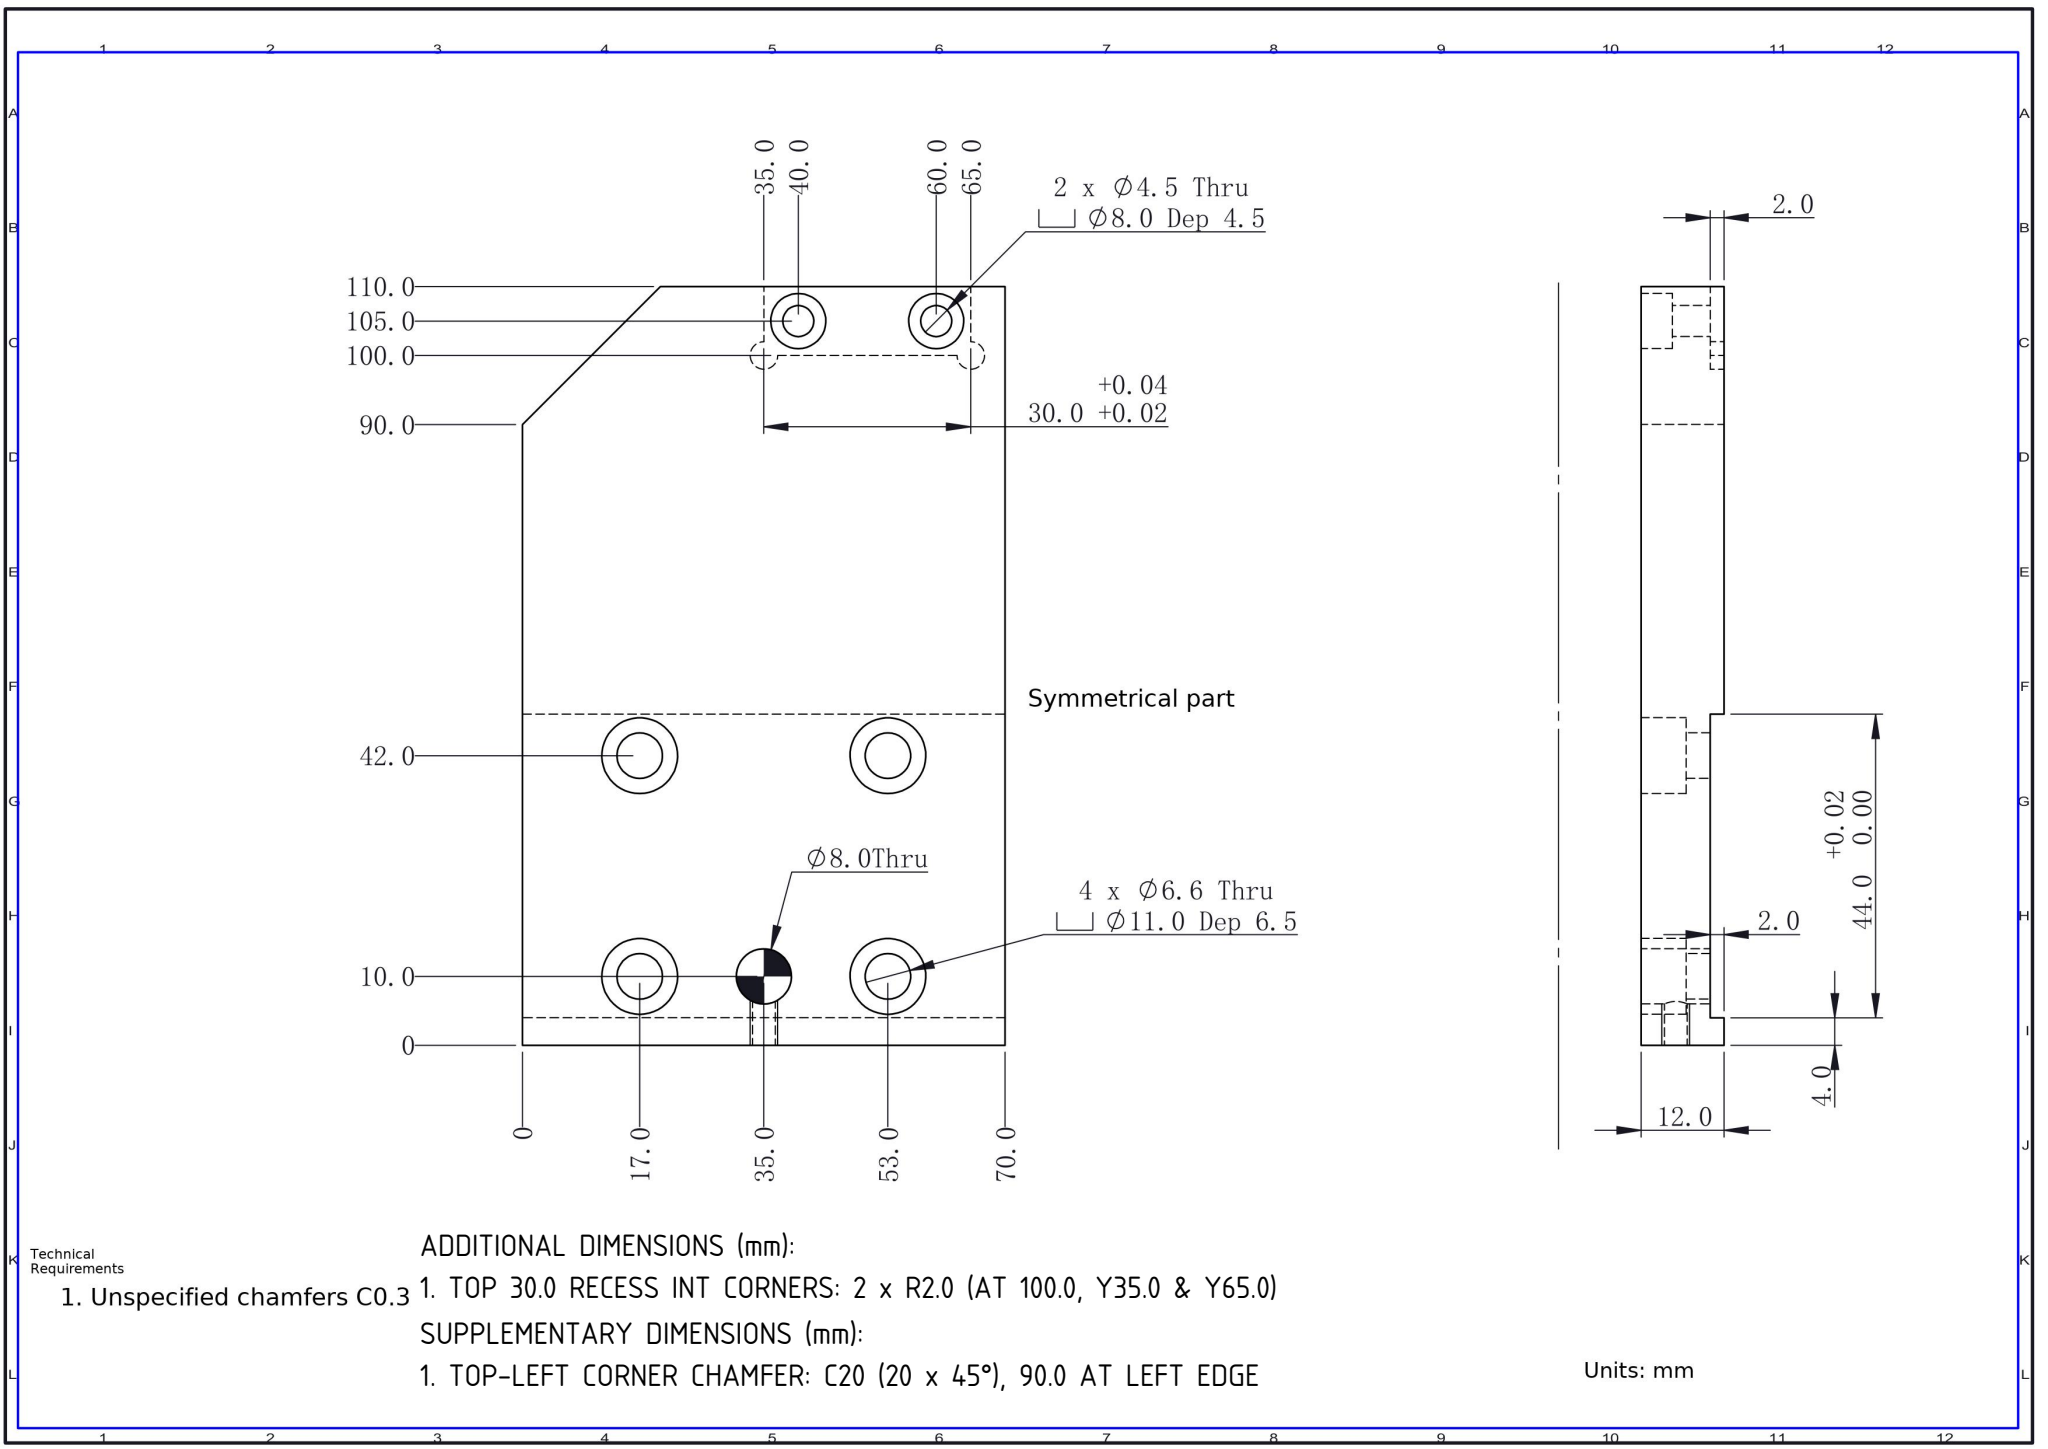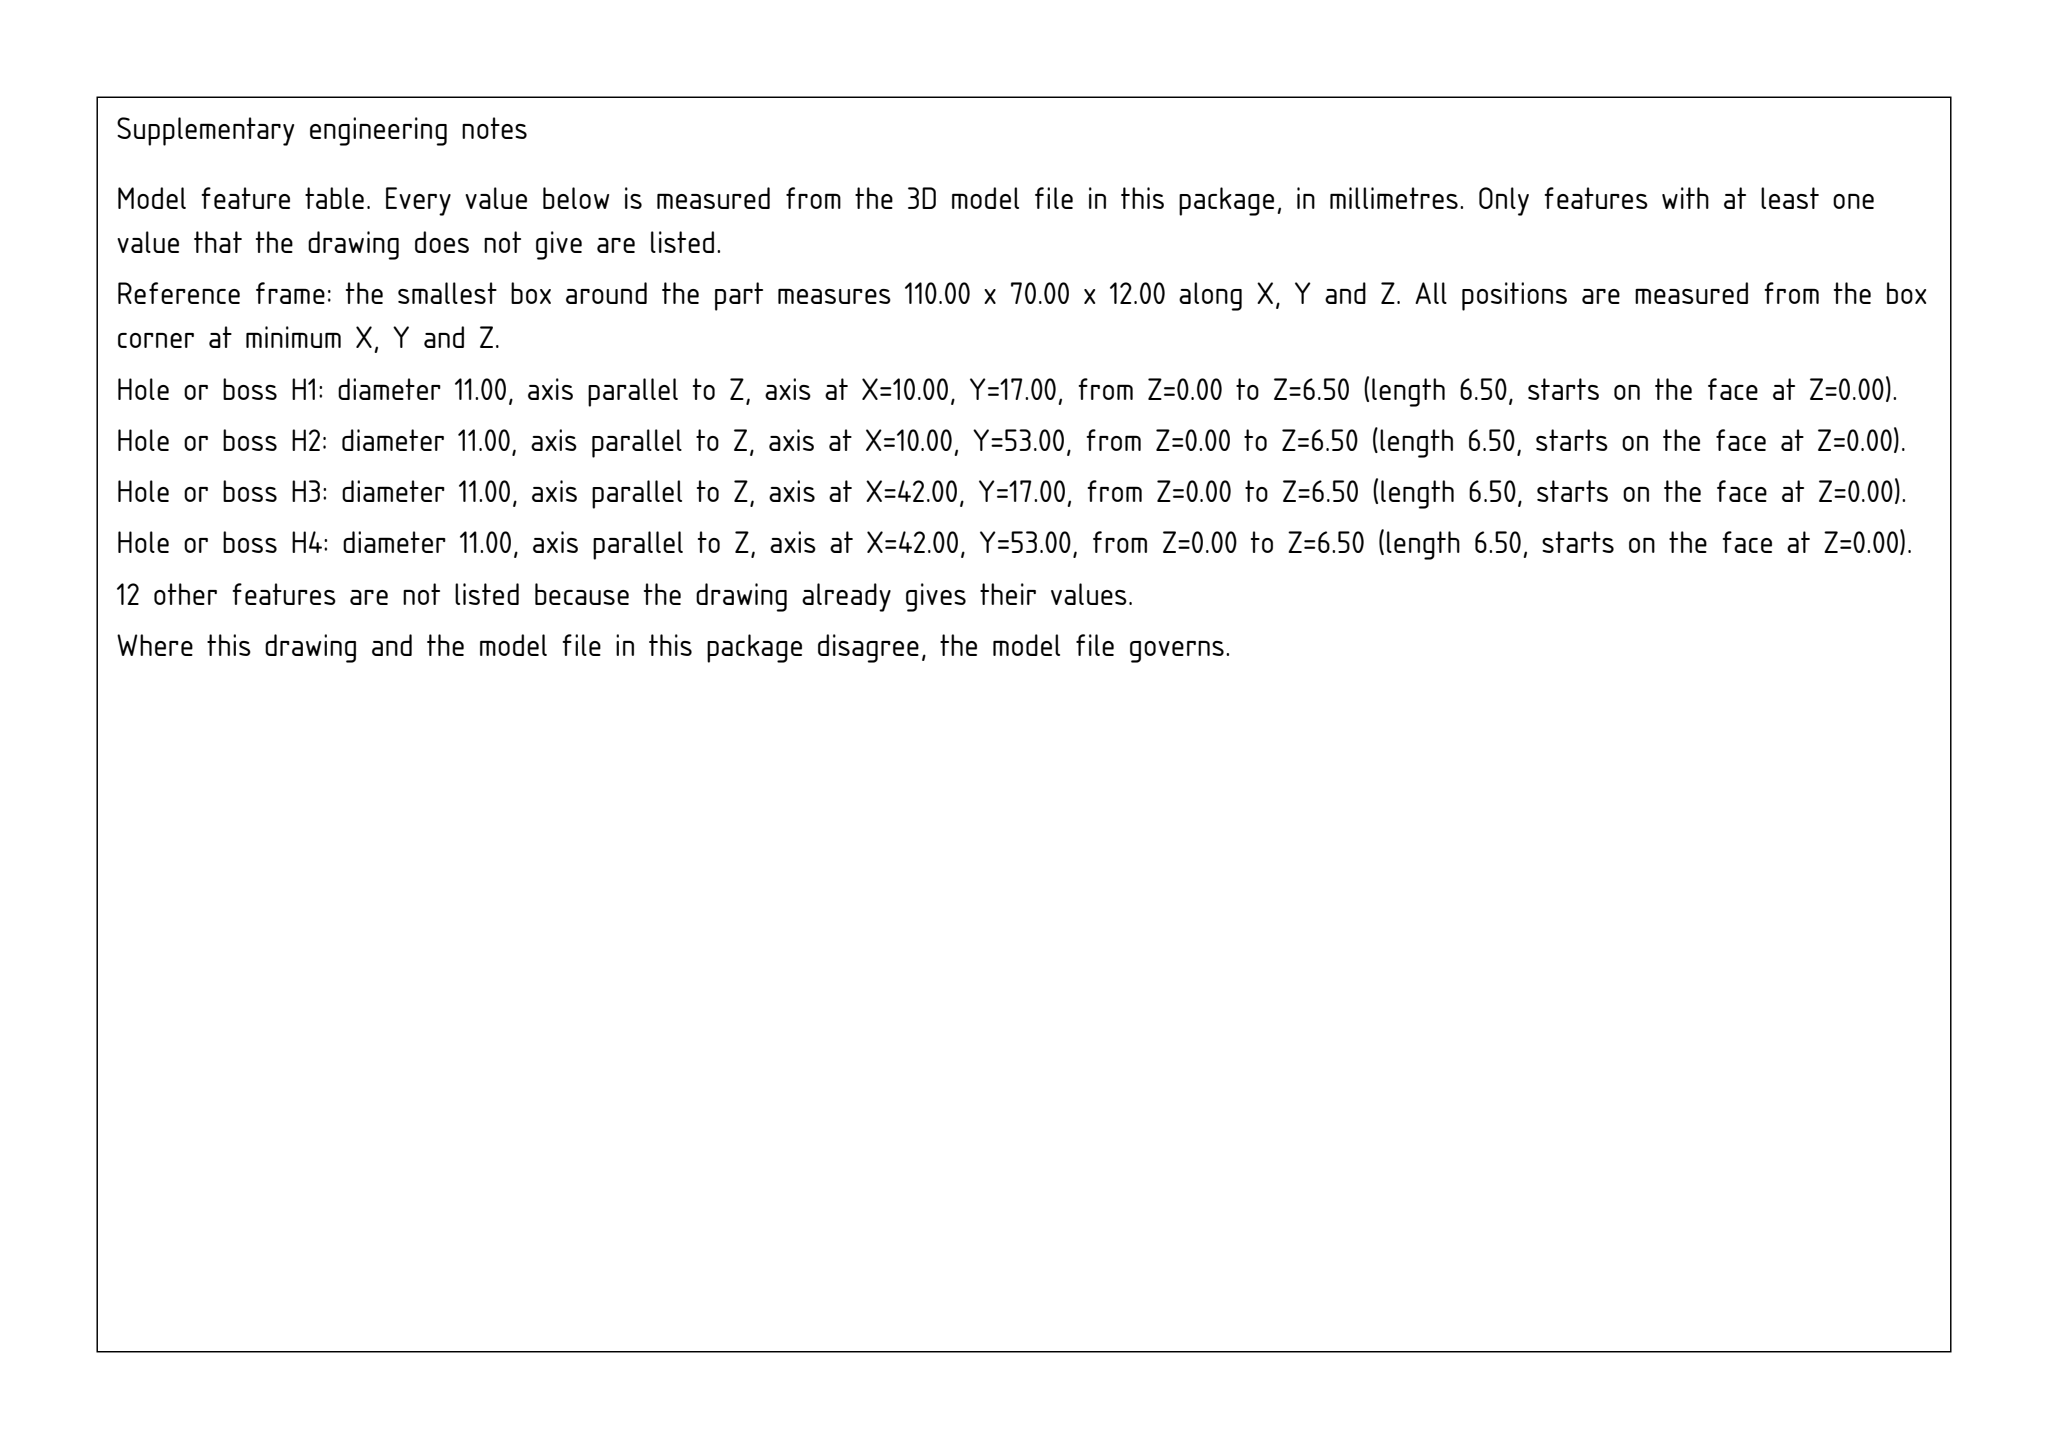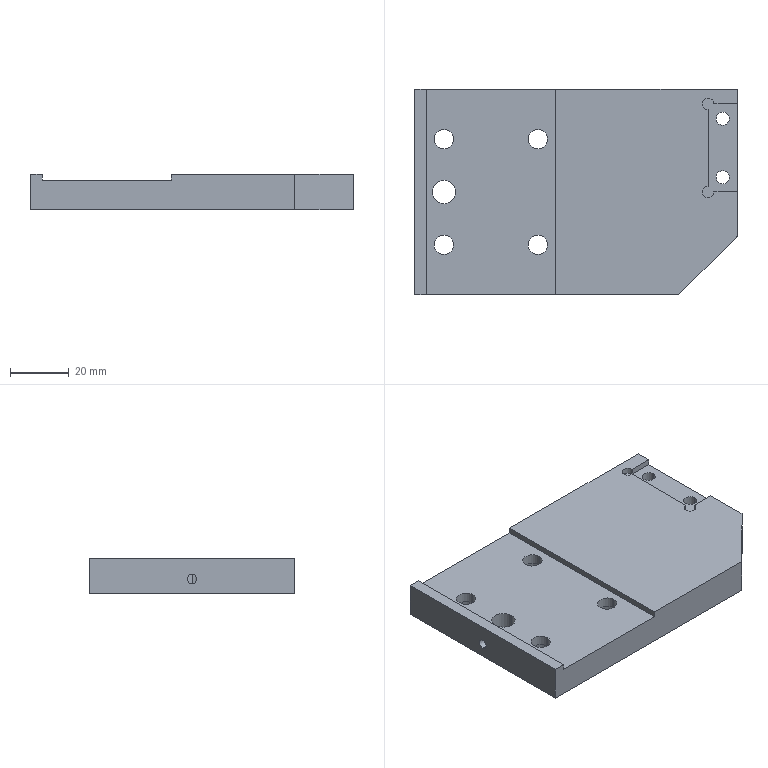Part | SolidWorks | mm | 1 solid | 51 faces | box 110 x 70 x 12 mm | volume 79070 mm3 | cylinder 30 | plane 21 | commonest cylinder face diameters 11 x8 6.6 x8 8 x6 4.5 x4 3.3 x2 4 x2
build123d program:
from build123d import *

# Parameters (mm, degrees)
SKETCH1_W                                       = 110
SKETCH1_H                                       = 70
BOSS_EXTRUDE1_DEPTH                             = 12
M6_HEX_SOCKET_HEAD_CAP_SCREW_CBORE1_D           = 6.6
M6_HEX_SOCKET_HEAD_CAP_SCREW_CBORE1_CBORE_D     = 11
M6_HEX_SOCKET_HEAD_CAP_SCREW_CBORE1_CBORE_DEPTH = 6.5
SKETCH6_W                                       = 44
SKETCH6_H                                       = 70
CUT_EXTRUDE1_DEPTH                              = 2
SIZE_MM_DOWEL_PIN_HOLE1_D                       = 8
SKETCH15_W                                      = 10
SKETCH15_H                                      = 30
CUT_EXTRUDE2_DEPTH                              = 2
SKETCH16_R                                      = 2
CUT_EXTRUDE3_DEPTH                              = 2
M4_HEX_SOCKET_HEAD_CAP_SCREW_CBORE1_D           = 4.5
M4_HEX_SOCKET_HEAD_CAP_SCREW_CBORE1_CBORE_D     = 8
M4_HEX_SOCKET_HEAD_CAP_SCREW_CBORE1_CBORE_DEPTH = 4.5
M4_TAPPED_HOLE1_REACH                           = 118.056
M4_TAPPED_HOLE1_BORE_R                          = 1.65
CHAMFER1_SIZE                                   = 20


with BuildPart() as part:
    # Sketch1 → Boss-Extrude1 (new body)
    with BuildSketch(Plane.XY):
        Rectangle(SKETCH1_W, SKETCH1_H)
    extrude(amount=BOSS_EXTRUDE1_DEPTH)

    # M6 Hex Socket Head Cap Screw CBORE1 (through all)
    with Locations(Plane(origin=(0, 0, 0), x_dir=(-1, 0, 0), z_dir=(0, 0, -1))):
        with Locations((13, -18), (13, 18), (45, 18), (45, -18)):
            CounterBoreHole(M6_HEX_SOCKET_HEAD_CAP_SCREW_CBORE1_D / 2, M6_HEX_SOCKET_HEAD_CAP_SCREW_CBORE1_CBORE_D / 2, M6_HEX_SOCKET_HEAD_CAP_SCREW_CBORE1_CBORE_DEPTH)

    # Sketch6 → Cut-Extrude1 (cut)
    with BuildSketch(Plane.XY.offset(12)):
        with Locations((-29, 0)):
            Rectangle(SKETCH6_W, SKETCH6_H)
    extrude(amount=-CUT_EXTRUDE1_DEPTH, mode=Mode.SUBTRACT)

    # Size mm Dowel Pin Hole1 (through all)
    with Locations(Plane(origin=(0, 0, 0), x_dir=(-1, 0, 0), z_dir=(0, 0, -1))):
        with Locations((45, 0)):
            Hole(SIZE_MM_DOWEL_PIN_HOLE1_D / 2)

    # Sketch15 → Cut-Extrude2 (cut)
    with BuildSketch(Plane.XY.offset(12)):
        with Locations((50, 15)):
            Rectangle(SKETCH15_W, SKETCH15_H)
    extrude(amount=-CUT_EXTRUDE2_DEPTH, mode=Mode.SUBTRACT)

    # Sketch16 → Cut-Extrude3 (cut)
    with BuildSketch(Plane.XY.offset(12)):
        with Locations((45, 30)):
            Circle(SKETCH16_R)
        with Locations((45, 0)):
            Circle(SKETCH16_R)
    extrude(amount=-CUT_EXTRUDE3_DEPTH, mode=Mode.SUBTRACT)

    # M4 Hex Socket Head Cap Screw CBORE1 (through all)
    with Locations(Plane(origin=(0, 0, 0), x_dir=(-1, 0, 0), z_dir=(0, 0, -1))):
        with Locations((-50, 5), (-50, 25)):
            CounterBoreHole(M4_HEX_SOCKET_HEAD_CAP_SCREW_CBORE1_D / 2, M4_HEX_SOCKET_HEAD_CAP_SCREW_CBORE1_CBORE_D / 2, M4_HEX_SOCKET_HEAD_CAP_SCREW_CBORE1_CBORE_DEPTH)

    # M4 Tapped Hole1 bore → M4 Tapped Hole1 (cut, up to next)
    with BuildSketch(Plane.ZY.offset(55), mode=Mode.PRIVATE) as m4_tapped_hole1_sk1:
        with Locations((5, 0)):
            Circle(M4_TAPPED_HOLE1_BORE_R)
    m4_tapped_hole1_tool1 = extrude(m4_tapped_hole1_sk1.sketch, amount=-M4_TAPPED_HOLE1_REACH, mode=Mode.PRIVATE) & part.part
    add(m4_tapped_hole1_tool1.solids().sort_by_distance((-55, 0, 5))[0], mode=Mode.SUBTRACT)

    # Chamfer1
    chamfer1_edges = [part.edges().sort_by_distance(p)[0] for p in [
        (55, -35, 6),
    ]]
    chamfer(chamfer1_edges, length=CHAMFER1_SIZE)


solid = part.part